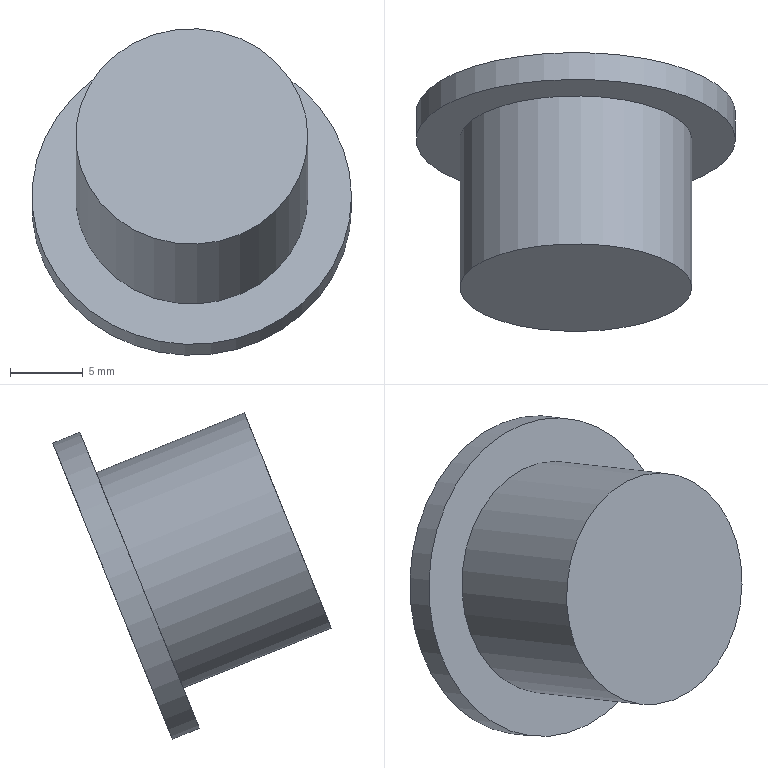Component | NX | 4 | 1 solid | 6 faces | box 22 x 19.17 x 22.49 mm | volume 1449 mm3 | plane 3 | cylinder 2 | sphere 1 | commonest cylinder face diameters 22 x1 16 x1
STEP:
#1=CARTESIAN_POINT('',(0.,0.,0.));
#2=DIRECTION('',(0.,0.,1.));
#3=DIRECTION('',(1.,0.,0.));
#4=AXIS2_PLACEMENT_3D('',#1,#2,#3);
#5=CARTESIAN_POINT('',(117.314,-110.934,-6.761));
#6=VERTEX_POINT('',#5);
#7=CARTESIAN_POINT('',(106.314,-110.934,-6.761));
#8=DIRECTION('',(0.,-0.9272,0.3746));
#9=DIRECTION('',(1.,0.,0.));
#10=AXIS2_PLACEMENT_3D('',#7,#8,#9);
#11=CIRCLE('',#10,11.);
#12=CARTESIAN_POINT('',(106.314,-110.934,-6.761));
#13=DIRECTION('',(0.,0.9272,-0.3746));
#14=DIRECTION('',(-1.,0.,0.));
#15=AXIS2_PLACEMENT_3D('',#12,#13,#14);
#16=CYLINDRICAL_SURFACE('',#15,11.);
#17=CARTESIAN_POINT('',(9.425,0.));
#18=DIRECTION('',(-1.,0.));
#19=VECTOR('',#18,1.);
#20=LINE('',#17,#19);
#21=(GEOMETRIC_REPRESENTATION_CONTEXT(2)PARAMETRIC_REPRESENTATION_CONTEXT()REPRESENTATION_CONTEXT('',''));
#22=DEFINITIONAL_REPRESENTATION('',(#20),#21);
#23=PCURVE('',#16,#22);
#24=CARTESIAN_POINT('',(106.314,-110.934,-6.761));
#25=DIRECTION('',(0.,-0.9272,0.3746));
#26=DIRECTION('',(1.,0.,0.));
#27=AXIS2_PLACEMENT_3D('',#24,#25,#26);
#28=PLANE('',#27);
#29=CARTESIAN_POINT('',(0.,0.));
#30=DIRECTION('',(1.,0.));
#31=AXIS2_PLACEMENT_2D('',#29,#30);
#32=CIRCLE('',#31,11.);
#33=(GEOMETRIC_REPRESENTATION_CONTEXT(2)PARAMETRIC_REPRESENTATION_CONTEXT()REPRESENTATION_CONTEXT('',''));
#34=DEFINITIONAL_REPRESENTATION('',(#32),#33);
#35=PCURVE('',#28,#34);
#36=SURFACE_CURVE('',#11,(#23,#35),.PCURVE_S1.);
#37=EDGE_CURVE('',#6,#6,#36,.T.);
#38=ORIENTED_EDGE('',*,*,#37,.F.);
#39=CARTESIAN_POINT('',(117.314,-109.079,-7.51));
#40=VERTEX_POINT('',#39);
#41=CARTESIAN_POINT('',(117.314,-110.934,-6.761));
#42=CARTESIAN_POINT('',(117.314,-109.079,-7.51));
#43=B_SPLINE_CURVE_WITH_KNOTS('',1,(#41,#42),.UNSPECIFIED.,.F.,.F.,(2,2),(0.,2.),.PIECEWISE_BEZIER_KNOTS.);
#44=CARTESIAN_POINT('',(9.425,0.));
#45=DIRECTION('',(0.,1.));
#46=VECTOR('',#45,1.);
#47=LINE('',#44,#46);
#48=(GEOMETRIC_REPRESENTATION_CONTEXT(2)PARAMETRIC_REPRESENTATION_CONTEXT()REPRESENTATION_CONTEXT('',''));
#49=DEFINITIONAL_REPRESENTATION('',(#47),#48);
#50=PCURVE('',#16,#49);
#51=CARTESIAN_POINT('',(3.142,0.));
#52=DIRECTION('',(0.,1.));
#53=VECTOR('',#52,1.);
#54=LINE('',#51,#53);
#55=(GEOMETRIC_REPRESENTATION_CONTEXT(2)PARAMETRIC_REPRESENTATION_CONTEXT()REPRESENTATION_CONTEXT('',''));
#56=DEFINITIONAL_REPRESENTATION('',(#54),#55);
#57=PCURVE('',#16,#56);
#58=SEAM_CURVE('',#43,(#50,#57),.PCURVE_S1.);
#59=EDGE_CURVE('',#6,#40,#58,.T.);
#60=ORIENTED_EDGE('',*,*,#59,.T.);
#61=CARTESIAN_POINT('',(106.314,-109.079,-7.51));
#62=DIRECTION('',(0.,-0.9272,0.3746));
#63=DIRECTION('',(1.,0.,0.));
#64=AXIS2_PLACEMENT_3D('',#61,#62,#63);
#65=CIRCLE('',#64,11.);
#66=CARTESIAN_POINT('',(9.425,2.));
#67=DIRECTION('',(-1.,0.));
#68=VECTOR('',#67,1.);
#69=LINE('',#66,#68);
#70=(GEOMETRIC_REPRESENTATION_CONTEXT(2)PARAMETRIC_REPRESENTATION_CONTEXT()REPRESENTATION_CONTEXT('',''));
#71=DEFINITIONAL_REPRESENTATION('',(#69),#70);
#72=PCURVE('',#16,#71);
#73=CARTESIAN_POINT('',(106.314,-109.079,-7.51));
#74=DIRECTION('',(0.,-0.9272,0.3746));
#75=DIRECTION('',(1.,0.,0.));
#76=AXIS2_PLACEMENT_3D('',#73,#74,#75);
#77=PLANE('',#76);
#78=CARTESIAN_POINT('',(0.,0.));
#79=DIRECTION('',(1.,0.));
#80=AXIS2_PLACEMENT_2D('',#78,#79);
#81=CIRCLE('',#80,11.);
#82=(GEOMETRIC_REPRESENTATION_CONTEXT(2)PARAMETRIC_REPRESENTATION_CONTEXT()REPRESENTATION_CONTEXT('',''));
#83=DEFINITIONAL_REPRESENTATION('',(#81),#82);
#84=PCURVE('',#77,#83);
#85=SURFACE_CURVE('',#65,(#72,#84),.PCURVE_S1.);
#86=EDGE_CURVE('',#40,#40,#85,.T.);
#87=ORIENTED_EDGE('',*,*,#86,.T.);
#88=ORIENTED_EDGE('',*,*,#59,.F.);
#89=EDGE_LOOP('',(#38,#60,#87,#88));
#90=FACE_BOUND('',#89,.T.);
#91=ADVANCED_FACE('',(#90),#16,.T.);
#92=CARTESIAN_POINT('',(114.314,-110.934,-6.761));
#93=VERTEX_POINT('',#92);
#94=CARTESIAN_POINT('',(106.314,-110.934,-6.761));
#95=DIRECTION('',(0.,-0.9272,0.3746));
#96=DIRECTION('',(1.,0.,0.));
#97=AXIS2_PLACEMENT_3D('',#94,#95,#96);
#98=CIRCLE('',#97,8.);
#99=CARTESIAN_POINT('',(0.,0.));
#100=DIRECTION('',(1.,0.));
#101=AXIS2_PLACEMENT_2D('',#99,#100);
#102=CIRCLE('',#101,8.);
#103=(GEOMETRIC_REPRESENTATION_CONTEXT(2)PARAMETRIC_REPRESENTATION_CONTEXT()REPRESENTATION_CONTEXT('',''));
#104=DEFINITIONAL_REPRESENTATION('',(#102),#103);
#105=PCURVE('',#28,#104);
#106=CARTESIAN_POINT('',(106.314,-121.133,-2.64));
#107=DIRECTION('',(0.,0.9272,-0.3746));
#108=DIRECTION('',(-1.,0.,0.));
#109=AXIS2_PLACEMENT_3D('',#106,#107,#108);
#110=CYLINDRICAL_SURFACE('',#109,8.);
#111=CARTESIAN_POINT('',(9.425,11.));
#112=DIRECTION('',(-1.,0.));
#113=VECTOR('',#112,1.);
#114=LINE('',#111,#113);
#115=(GEOMETRIC_REPRESENTATION_CONTEXT(2)PARAMETRIC_REPRESENTATION_CONTEXT()REPRESENTATION_CONTEXT('',''));
#116=DEFINITIONAL_REPRESENTATION('',(#114),#115);
#117=PCURVE('',#110,#116);
#118=SURFACE_CURVE('',#98,(#105,#117),.PCURVE_S1.);
#119=EDGE_CURVE('',#93,#93,#118,.T.);
#120=ORIENTED_EDGE('',*,*,#119,.F.);
#121=EDGE_LOOP('',(#120));
#122=FACE_BOUND('',#121,.T.);
#123=ORIENTED_EDGE('',*,*,#37,.T.);
#124=EDGE_LOOP('',(#123));
#125=FACE_BOUND('',#124,.T.);
#126=ADVANCED_FACE('',(#122,#125),#28,.T.);
#127=CARTESIAN_POINT('',(112.658,-109.079,-7.51));
#128=VERTEX_POINT('',#127);
#129=CARTESIAN_POINT('',(106.314,-109.079,-7.51));
#130=DIRECTION('',(0.,-0.9272,0.3746));
#131=DIRECTION('',(1.,0.,0.));
#132=AXIS2_PLACEMENT_3D('',#129,#130,#131);
#133=CIRCLE('',#132,6.344);
#134=CARTESIAN_POINT('',(0.,0.));
#135=DIRECTION('',(1.,0.));
#136=AXIS2_PLACEMENT_2D('',#134,#135);
#137=CIRCLE('',#136,6.344);
#138=(GEOMETRIC_REPRESENTATION_CONTEXT(2)PARAMETRIC_REPRESENTATION_CONTEXT()REPRESENTATION_CONTEXT('',''));
#139=DEFINITIONAL_REPRESENTATION('',(#137),#138);
#140=PCURVE('',#77,#139);
#141=CARTESIAN_POINT('',(106.314,-112.788,-6.012));
#142=DIRECTION('',(0.,-0.9272,0.3746));
#143=DIRECTION('',(1.,0.,0.));
#144=AXIS2_PLACEMENT_3D('',#141,#142,#143);
#145=SPHERICAL_SURFACE('',#144,7.5);
#146=CARTESIAN_POINT('',(-0.,-0.5625));
#147=CARTESIAN_POINT('',(0.0952,-0.5625));
#148=CARTESIAN_POINT('',(0.2856,-0.5625));
#149=CARTESIAN_POINT('',(0.5712,-0.5625));
#150=CARTESIAN_POINT('',(0.8568,-0.5625));
#151=CARTESIAN_POINT('',(1.142,-0.5625));
#152=CARTESIAN_POINT('',(1.428,-0.5625));
#153=CARTESIAN_POINT('',(1.714,-0.5625));
#154=CARTESIAN_POINT('',(1.999,-0.5625));
#155=CARTESIAN_POINT('',(2.285,-0.5625));
#156=CARTESIAN_POINT('',(2.57,-0.5625));
#157=CARTESIAN_POINT('',(2.856,-0.5625));
#158=CARTESIAN_POINT('',(3.142,-0.5625));
#159=CARTESIAN_POINT('',(3.427,-0.5625));
#160=CARTESIAN_POINT('',(3.713,-0.5625));
#161=CARTESIAN_POINT('',(3.998,-0.5625));
#162=CARTESIAN_POINT('',(4.284,-0.5625));
#163=CARTESIAN_POINT('',(4.57,-0.5625));
#164=CARTESIAN_POINT('',(4.855,-0.5625));
#165=CARTESIAN_POINT('',(5.141,-0.5625));
#166=CARTESIAN_POINT('',(5.426,-0.5625));
#167=CARTESIAN_POINT('',(5.712,-0.5625));
#168=CARTESIAN_POINT('',(5.998,-0.5625));
#169=CARTESIAN_POINT('',(6.188,-0.5625));
#170=CARTESIAN_POINT('',(6.283,-0.5625));
#171=B_SPLINE_CURVE_WITH_KNOTS('',3,(#146,#147,#148,#149,#150,#151,#152,#153,#154,#155,#156,#157,#158,#159,#160,#161,#162,#163,#164,#165,#166,#167,#168,#169,#170),.UNSPECIFIED.,.F.,.F.,(4,1,1,1,1,1,1,1,1,1,1,1,1,1,1,1,1,1,1,1,1,1,4),(0.,0.2856,0.5712,0.8568,1.142,1.428,1.714,1.999,2.285,2.57,2.856,3.142,3.427,3.713,3.998,4.284,4.57,4.855,5.141,5.426,5.712,5.998,6.283),.QUASI_UNIFORM_KNOTS.);
#172=(GEOMETRIC_REPRESENTATION_CONTEXT(2)PARAMETRIC_REPRESENTATION_CONTEXT()REPRESENTATION_CONTEXT('',''));
#173=DEFINITIONAL_REPRESENTATION('',(#171),#172);
#174=PCURVE('',#145,#173);
#175=SURFACE_CURVE('',#133,(#140,#174),.PCURVE_S1.);
#176=EDGE_CURVE('',#128,#128,#175,.T.);
#177=ORIENTED_EDGE('',*,*,#176,.T.);
#178=EDGE_LOOP('',(#177));
#179=FACE_BOUND('',#178,.T.);
#180=ORIENTED_EDGE('',*,*,#86,.F.);
#181=EDGE_LOOP('',(#180));
#182=FACE_BOUND('',#181,.T.);
#183=ADVANCED_FACE('',(#179,#182),#77,.F.);
#184=CARTESIAN_POINT('',(114.314,-121.133,-2.64));
#185=VERTEX_POINT('',#184);
#186=CARTESIAN_POINT('',(106.314,-121.133,-2.64));
#187=DIRECTION('',(0.,-0.9272,0.3746));
#188=DIRECTION('',(1.,0.,0.));
#189=AXIS2_PLACEMENT_3D('',#186,#187,#188);
#190=CIRCLE('',#189,8.);
#191=CARTESIAN_POINT('',(9.425,0.));
#192=DIRECTION('',(-1.,0.));
#193=VECTOR('',#192,1.);
#194=LINE('',#191,#193);
#195=(GEOMETRIC_REPRESENTATION_CONTEXT(2)PARAMETRIC_REPRESENTATION_CONTEXT()REPRESENTATION_CONTEXT('',''));
#196=DEFINITIONAL_REPRESENTATION('',(#194),#195);
#197=PCURVE('',#110,#196);
#198=CARTESIAN_POINT('',(106.314,-121.133,-2.64));
#199=DIRECTION('',(0.,-0.9272,0.3746));
#200=DIRECTION('',(1.,0.,0.));
#201=AXIS2_PLACEMENT_3D('',#198,#199,#200);
#202=PLANE('',#201);
#203=CARTESIAN_POINT('',(0.,0.));
#204=DIRECTION('',(1.,0.));
#205=AXIS2_PLACEMENT_2D('',#203,#204);
#206=CIRCLE('',#205,8.);
#207=(GEOMETRIC_REPRESENTATION_CONTEXT(2)PARAMETRIC_REPRESENTATION_CONTEXT()REPRESENTATION_CONTEXT('',''));
#208=DEFINITIONAL_REPRESENTATION('',(#206),#207);
#209=PCURVE('',#202,#208);
#210=SURFACE_CURVE('',#190,(#197,#209),.PCURVE_S1.);
#211=EDGE_CURVE('',#185,#185,#210,.T.);
#212=ORIENTED_EDGE('',*,*,#211,.F.);
#213=CARTESIAN_POINT('',(114.314,-121.133,-2.64));
#214=CARTESIAN_POINT('',(114.314,-110.934,-6.761));
#215=B_SPLINE_CURVE_WITH_KNOTS('',1,(#213,#214),.UNSPECIFIED.,.F.,.F.,(2,2),(0.,11.),.PIECEWISE_BEZIER_KNOTS.);
#216=CARTESIAN_POINT('',(9.425,0.));
#217=DIRECTION('',(0.,1.));
#218=VECTOR('',#217,1.);
#219=LINE('',#216,#218);
#220=(GEOMETRIC_REPRESENTATION_CONTEXT(2)PARAMETRIC_REPRESENTATION_CONTEXT()REPRESENTATION_CONTEXT('',''));
#221=DEFINITIONAL_REPRESENTATION('',(#219),#220);
#222=PCURVE('',#110,#221);
#223=CARTESIAN_POINT('',(3.142,0.));
#224=DIRECTION('',(0.,1.));
#225=VECTOR('',#224,1.);
#226=LINE('',#223,#225);
#227=(GEOMETRIC_REPRESENTATION_CONTEXT(2)PARAMETRIC_REPRESENTATION_CONTEXT()REPRESENTATION_CONTEXT('',''));
#228=DEFINITIONAL_REPRESENTATION('',(#226),#227);
#229=PCURVE('',#110,#228);
#230=SEAM_CURVE('',#215,(#222,#229),.PCURVE_S1.);
#231=EDGE_CURVE('',#185,#93,#230,.T.);
#232=ORIENTED_EDGE('',*,*,#231,.T.);
#233=ORIENTED_EDGE('',*,*,#119,.T.);
#234=ORIENTED_EDGE('',*,*,#231,.F.);
#235=EDGE_LOOP('',(#212,#232,#233,#234));
#236=FACE_BOUND('',#235,.T.);
#237=ADVANCED_FACE('',(#236),#110,.T.);
#238=ORIENTED_EDGE('',*,*,#211,.T.);
#239=EDGE_LOOP('',(#238));
#240=FACE_BOUND('',#239,.T.);
#241=ADVANCED_FACE('',(#240),#202,.T.);
#242=ORIENTED_EDGE('',*,*,#176,.T.);
#243=CARTESIAN_POINT('',(106.314,-119.742,-3.202));
#244=VERTEX_POINT('',#243);
#245=CARTESIAN_POINT('',(112.658,-109.079,-7.51));
#246=CARTESIAN_POINT('',(113.877,-110.872,-6.786));
#247=CARTESIAN_POINT('',(114.409,-113.067,-5.899));
#248=CARTESIAN_POINT('',(114.069,-115.391,-4.96));
#249=CARTESIAN_POINT('',(112.825,-117.482,-4.116));
#250=CARTESIAN_POINT('',(110.885,-118.989,-3.507));
#251=CARTESIAN_POINT('',(108.6,-119.742,-3.202));
#252=CARTESIAN_POINT('',(106.314,-119.742,-3.202));
#253=B_SPLINE_CURVE_WITH_KNOTS('',7,(#245,#246,#247,#248,#249,#250,#251,#252),.UNSPECIFIED.,.F.,.F.,(8,8),(-0.5625,1.571),.PIECEWISE_BEZIER_KNOTS.);
#254=CARTESIAN_POINT('',(6.283,0.));
#255=DIRECTION('',(0.,1.));
#256=VECTOR('',#255,1.);
#257=LINE('',#254,#256);
#258=(GEOMETRIC_REPRESENTATION_CONTEXT(2)PARAMETRIC_REPRESENTATION_CONTEXT()REPRESENTATION_CONTEXT('',''));
#259=DEFINITIONAL_REPRESENTATION('',(#257),#258);
#260=PCURVE('',#145,#259);
#261=CARTESIAN_POINT('',(-0.,0.));
#262=DIRECTION('',(0.,1.));
#263=VECTOR('',#262,1.);
#264=LINE('',#261,#263);
#265=(GEOMETRIC_REPRESENTATION_CONTEXT(2)PARAMETRIC_REPRESENTATION_CONTEXT()REPRESENTATION_CONTEXT('',''));
#266=DEFINITIONAL_REPRESENTATION('',(#264),#265);
#267=PCURVE('',#145,#266);
#268=SEAM_CURVE('',#253,(#260,#267),.PCURVE_S1.);
#269=EDGE_CURVE('',#128,#244,#268,.T.);
#270=ORIENTED_EDGE('',*,*,#269,.T.);
#271=ORIENTED_EDGE('',*,*,#269,.F.);
#272=EDGE_LOOP('',(#242,#270,#271));
#273=FACE_BOUND('',#272,.F.);
#274=ADVANCED_FACE('',(#273),#145,.F.);
#275=CLOSED_SHELL('',(#91,#126,#183,#237,#241,#274));
#276=MANIFOLD_SOLID_BREP('',#275);
#277=(LENGTH_UNIT()NAMED_UNIT(*)SI_UNIT(.MILLI.,.METRE.));
#278=UNCERTAINTY_MEASURE_WITH_UNIT(LENGTH_MEASURE(0.00001),#277,'','');
#279=(NAMED_UNIT(*)PLANE_ANGLE_UNIT()SI_UNIT($,.RADIAN.));
#280=(NAMED_UNIT(*)SI_UNIT($,.STERADIAN.)SOLID_ANGLE_UNIT());
#281=(GEOMETRIC_REPRESENTATION_CONTEXT(3)GLOBAL_UNCERTAINTY_ASSIGNED_CONTEXT((#278))GLOBAL_UNIT_ASSIGNED_CONTEXT((#277,#279,#280))REPRESENTATION_CONTEXT('',''));
#282=ADVANCED_BREP_SHAPE_REPRESENTATION('',(#4,#276),#281);